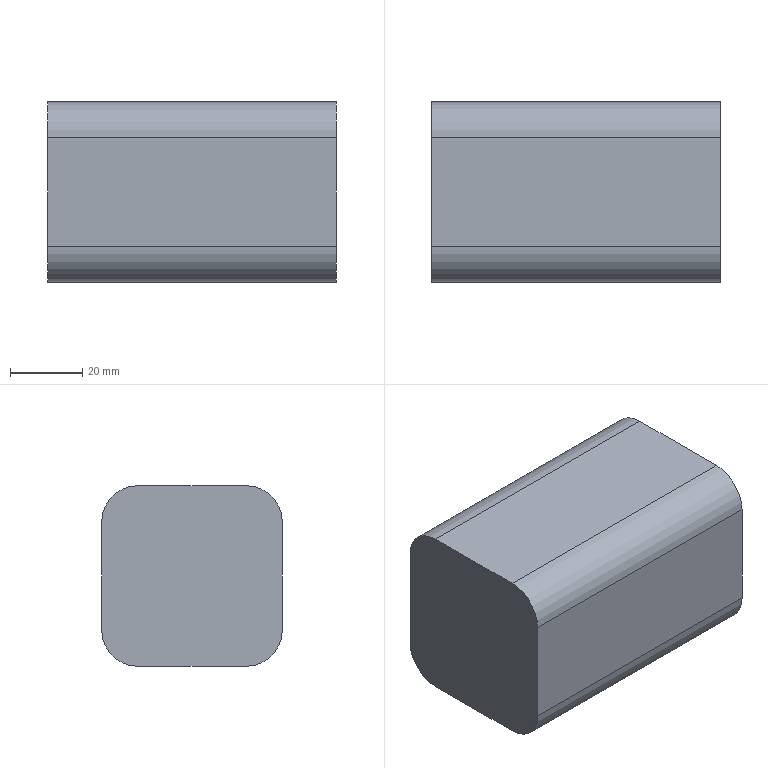Component | NX | MOTOR | 1 solid | 12 faces | box 80 x 50 x 50 mm | volume 187831 mm3 | plane 7 | cylinder 5 | commonest cylinder face diameters 20 x4 15 x1
STEP:
#1=CARTESIAN_POINT('',(0.,0.,0.));
#2=DIRECTION('',(0.,0.,1.));
#3=DIRECTION('',(1.,0.,0.));
#4=AXIS2_PLACEMENT_3D('',#1,#2,#3);
#5=CARTESIAN_POINT('',(213.574,526.538,-180.));
#6=VERTEX_POINT('',#5);
#7=CARTESIAN_POINT('',(213.574,526.538,-210.));
#8=VERTEX_POINT('',#7);
#9=CARTESIAN_POINT('',(213.574,526.538,-180.));
#10=DIRECTION('',(0.,0.,-1.));
#11=VECTOR('',#10,1.);
#12=LINE('',#9,#11);
#13=CARTESIAN_POINT('',(133.574,526.538,-180.));
#14=DIRECTION('',(0.,-1.,0.));
#15=DIRECTION('',(0.,0.,-1.));
#16=AXIS2_PLACEMENT_3D('',#13,#14,#15);
#17=PLANE('',#16);
#18=CARTESIAN_POINT('',(0.,80.));
#19=DIRECTION('',(1.,0.));
#20=VECTOR('',#19,1.);
#21=LINE('',#18,#20);
#22=(GEOMETRIC_REPRESENTATION_CONTEXT(2)PARAMETRIC_REPRESENTATION_CONTEXT()REPRESENTATION_CONTEXT('',''));
#23=DEFINITIONAL_REPRESENTATION('',(#21),#22);
#24=PCURVE('',#17,#23);
#25=CARTESIAN_POINT('',(213.574,516.538,-210.));
#26=DIRECTION('',(-1.,0.,0.));
#27=DIRECTION('',(0.,0.,-1.));
#28=AXIS2_PLACEMENT_3D('',#25,#26,#27);
#29=PLANE('',#28);
#30=CARTESIAN_POINT('',(-30.,-10.));
#31=DIRECTION('',(1.,0.));
#32=VECTOR('',#31,1.);
#33=LINE('',#30,#32);
#34=(GEOMETRIC_REPRESENTATION_CONTEXT(2)PARAMETRIC_REPRESENTATION_CONTEXT()REPRESENTATION_CONTEXT('',''));
#35=DEFINITIONAL_REPRESENTATION('',(#33),#34);
#36=PCURVE('',#29,#35);
#37=SURFACE_CURVE('',#12,(#24,#36),.PCURVE_S1.);
#38=EDGE_CURVE('',#6,#8,#37,.T.);
#39=ORIENTED_EDGE('',*,*,#38,.T.);
#40=CARTESIAN_POINT('',(133.574,526.538,-210.));
#41=VERTEX_POINT('',#40);
#42=CARTESIAN_POINT('',(133.574,526.538,-210.));
#43=DIRECTION('',(1.,0.,0.));
#44=VECTOR('',#43,1.);
#45=LINE('',#42,#44);
#46=CARTESIAN_POINT('',(30.,0.));
#47=DIRECTION('',(0.,1.));
#48=VECTOR('',#47,1.);
#49=LINE('',#46,#48);
#50=(GEOMETRIC_REPRESENTATION_CONTEXT(2)PARAMETRIC_REPRESENTATION_CONTEXT()REPRESENTATION_CONTEXT('',''));
#51=DEFINITIONAL_REPRESENTATION('',(#49),#50);
#52=PCURVE('',#17,#51);
#53=CARTESIAN_POINT('',(133.574,516.538,-210.));
#54=DIRECTION('',(1.,0.,0.));
#55=DIRECTION('',(0.,0.,1.));
#56=AXIS2_PLACEMENT_3D('',#53,#54,#55);
#57=CYLINDRICAL_SURFACE('',#56,10.);
#58=CARTESIAN_POINT('',(4.712,0.));
#59=DIRECTION('',(0.,1.));
#60=VECTOR('',#59,1.);
#61=LINE('',#58,#60);
#62=(GEOMETRIC_REPRESENTATION_CONTEXT(2)PARAMETRIC_REPRESENTATION_CONTEXT()REPRESENTATION_CONTEXT('',''));
#63=DEFINITIONAL_REPRESENTATION('',(#61),#62);
#64=PCURVE('',#57,#63);
#65=SURFACE_CURVE('',#45,(#52,#64),.PCURVE_S1.);
#66=EDGE_CURVE('',#41,#8,#65,.T.);
#67=ORIENTED_EDGE('',*,*,#66,.F.);
#68=CARTESIAN_POINT('',(133.574,526.538,-180.));
#69=VERTEX_POINT('',#68);
#70=CARTESIAN_POINT('',(133.574,526.538,-180.));
#71=DIRECTION('',(0.,0.,-1.));
#72=VECTOR('',#71,1.);
#73=LINE('',#70,#72);
#74=CARTESIAN_POINT('',(0.,0.));
#75=DIRECTION('',(1.,0.));
#76=VECTOR('',#75,1.);
#77=LINE('',#74,#76);
#78=(GEOMETRIC_REPRESENTATION_CONTEXT(2)PARAMETRIC_REPRESENTATION_CONTEXT()REPRESENTATION_CONTEXT('',''));
#79=DEFINITIONAL_REPRESENTATION('',(#77),#78);
#80=PCURVE('',#17,#79);
#81=CARTESIAN_POINT('',(133.574,516.538,-210.));
#82=DIRECTION('',(-1.,0.,0.));
#83=DIRECTION('',(0.,0.,-1.));
#84=AXIS2_PLACEMENT_3D('',#81,#82,#83);
#85=PLANE('',#84);
#86=CARTESIAN_POINT('',(-30.,-10.));
#87=DIRECTION('',(1.,0.));
#88=VECTOR('',#87,1.);
#89=LINE('',#86,#88);
#90=(GEOMETRIC_REPRESENTATION_CONTEXT(2)PARAMETRIC_REPRESENTATION_CONTEXT()REPRESENTATION_CONTEXT('',''));
#91=DEFINITIONAL_REPRESENTATION('',(#89),#90);
#92=PCURVE('',#85,#91);
#93=SURFACE_CURVE('',#73,(#80,#92),.PCURVE_S1.);
#94=EDGE_CURVE('',#69,#41,#93,.T.);
#95=ORIENTED_EDGE('',*,*,#94,.F.);
#96=CARTESIAN_POINT('',(133.574,526.538,-180.));
#97=DIRECTION('',(1.,0.,0.));
#98=VECTOR('',#97,1.);
#99=LINE('',#96,#98);
#100=CARTESIAN_POINT('',(0.,0.));
#101=DIRECTION('',(0.,1.));
#102=VECTOR('',#101,1.);
#103=LINE('',#100,#102);
#104=(GEOMETRIC_REPRESENTATION_CONTEXT(2)PARAMETRIC_REPRESENTATION_CONTEXT()REPRESENTATION_CONTEXT('',''));
#105=DEFINITIONAL_REPRESENTATION('',(#103),#104);
#106=PCURVE('',#17,#105);
#107=CARTESIAN_POINT('',(133.574,516.538,-180.));
#108=DIRECTION('',(1.,0.,0.));
#109=DIRECTION('',(0.,0.,1.));
#110=AXIS2_PLACEMENT_3D('',#107,#108,#109);
#111=CYLINDRICAL_SURFACE('',#110,10.);
#112=CARTESIAN_POINT('',(4.712,0.));
#113=DIRECTION('',(0.,1.));
#114=VECTOR('',#113,1.);
#115=LINE('',#112,#114);
#116=(GEOMETRIC_REPRESENTATION_CONTEXT(2)PARAMETRIC_REPRESENTATION_CONTEXT()REPRESENTATION_CONTEXT('',''));
#117=DEFINITIONAL_REPRESENTATION('',(#115),#116);
#118=PCURVE('',#111,#117);
#119=SURFACE_CURVE('',#99,(#106,#118),.PCURVE_S1.);
#120=EDGE_CURVE('',#69,#6,#119,.T.);
#121=ORIENTED_EDGE('',*,*,#120,.T.);
#122=EDGE_LOOP('',(#39,#67,#95,#121));
#123=FACE_BOUND('',#122,.T.);
#124=ADVANCED_FACE('',(#123),#17,.F.);
#125=CARTESIAN_POINT('',(213.574,516.538,-220.));
#126=VERTEX_POINT('',#125);
#127=CARTESIAN_POINT('',(213.574,516.538,-210.));
#128=DIRECTION('',(-1.,0.,0.));
#129=DIRECTION('',(0.,-1.,0.));
#130=AXIS2_PLACEMENT_3D('',#127,#128,#129);
#131=CIRCLE('',#130,10.);
#132=CARTESIAN_POINT('',(7.854,80.));
#133=DIRECTION('',(-1.,0.));
#134=VECTOR('',#133,1.);
#135=LINE('',#132,#134);
#136=(GEOMETRIC_REPRESENTATION_CONTEXT(2)PARAMETRIC_REPRESENTATION_CONTEXT()REPRESENTATION_CONTEXT('',''));
#137=DEFINITIONAL_REPRESENTATION('',(#135),#136);
#138=PCURVE('',#57,#137);
#139=CARTESIAN_POINT('',(0.,0.));
#140=DIRECTION('',(0.,1.));
#141=AXIS2_PLACEMENT_2D('',#139,#140);
#142=CIRCLE('',#141,10.);
#143=(GEOMETRIC_REPRESENTATION_CONTEXT(2)PARAMETRIC_REPRESENTATION_CONTEXT()REPRESENTATION_CONTEXT('',''));
#144=DEFINITIONAL_REPRESENTATION('',(#142),#143);
#145=PCURVE('',#29,#144);
#146=SURFACE_CURVE('',#131,(#138,#145),.PCURVE_S1.);
#147=EDGE_CURVE('',#8,#126,#146,.T.);
#148=ORIENTED_EDGE('',*,*,#147,.T.);
#149=CARTESIAN_POINT('',(133.574,516.538,-220.));
#150=VERTEX_POINT('',#149);
#151=CARTESIAN_POINT('',(133.574,516.538,-220.));
#152=DIRECTION('',(1.,0.,0.));
#153=VECTOR('',#152,1.);
#154=LINE('',#151,#153);
#155=CARTESIAN_POINT('',(3.142,0.));
#156=DIRECTION('',(0.,1.));
#157=VECTOR('',#156,1.);
#158=LINE('',#155,#157);
#159=(GEOMETRIC_REPRESENTATION_CONTEXT(2)PARAMETRIC_REPRESENTATION_CONTEXT()REPRESENTATION_CONTEXT('',''));
#160=DEFINITIONAL_REPRESENTATION('',(#158),#159);
#161=PCURVE('',#57,#160);
#162=CARTESIAN_POINT('',(133.574,516.538,-220.));
#163=DIRECTION('',(0.,-0.,1.));
#164=DIRECTION('',(0.,-1.,-0.));
#165=AXIS2_PLACEMENT_3D('',#162,#163,#164);
#166=PLANE('',#165);
#167=CARTESIAN_POINT('',(0.,0.));
#168=DIRECTION('',(0.,1.));
#169=VECTOR('',#168,1.);
#170=LINE('',#167,#169);
#171=(GEOMETRIC_REPRESENTATION_CONTEXT(2)PARAMETRIC_REPRESENTATION_CONTEXT()REPRESENTATION_CONTEXT('',''));
#172=DEFINITIONAL_REPRESENTATION('',(#170),#171);
#173=PCURVE('',#166,#172);
#174=SURFACE_CURVE('',#154,(#161,#173),.PCURVE_S1.);
#175=EDGE_CURVE('',#150,#126,#174,.T.);
#176=ORIENTED_EDGE('',*,*,#175,.F.);
#177=CARTESIAN_POINT('',(133.574,516.538,-210.));
#178=DIRECTION('',(-1.,0.,0.));
#179=DIRECTION('',(0.,-1.,0.));
#180=AXIS2_PLACEMENT_3D('',#177,#178,#179);
#181=CIRCLE('',#180,10.);
#182=CARTESIAN_POINT('',(7.854,0.));
#183=DIRECTION('',(-1.,0.));
#184=VECTOR('',#183,1.);
#185=LINE('',#182,#184);
#186=(GEOMETRIC_REPRESENTATION_CONTEXT(2)PARAMETRIC_REPRESENTATION_CONTEXT()REPRESENTATION_CONTEXT('',''));
#187=DEFINITIONAL_REPRESENTATION('',(#185),#186);
#188=PCURVE('',#57,#187);
#189=CARTESIAN_POINT('',(0.,0.));
#190=DIRECTION('',(0.,1.));
#191=AXIS2_PLACEMENT_2D('',#189,#190);
#192=CIRCLE('',#191,10.);
#193=(GEOMETRIC_REPRESENTATION_CONTEXT(2)PARAMETRIC_REPRESENTATION_CONTEXT()REPRESENTATION_CONTEXT('',''));
#194=DEFINITIONAL_REPRESENTATION('',(#192),#193);
#195=PCURVE('',#85,#194);
#196=SURFACE_CURVE('',#181,(#188,#195),.PCURVE_S1.);
#197=EDGE_CURVE('',#41,#150,#196,.T.);
#198=ORIENTED_EDGE('',*,*,#197,.F.);
#199=ORIENTED_EDGE('',*,*,#66,.T.);
#200=EDGE_LOOP('',(#148,#176,#198,#199));
#201=FACE_BOUND('',#200,.T.);
#202=ADVANCED_FACE('',(#201),#57,.T.);
#203=CARTESIAN_POINT('',(213.574,486.538,-220.));
#204=VERTEX_POINT('',#203);
#205=CARTESIAN_POINT('',(213.574,516.538,-220.));
#206=DIRECTION('',(0.,-1.,-0.));
#207=VECTOR('',#206,1.);
#208=LINE('',#205,#207);
#209=CARTESIAN_POINT('',(0.,80.));
#210=DIRECTION('',(1.,0.));
#211=VECTOR('',#210,1.);
#212=LINE('',#209,#211);
#213=(GEOMETRIC_REPRESENTATION_CONTEXT(2)PARAMETRIC_REPRESENTATION_CONTEXT()REPRESENTATION_CONTEXT('',''));
#214=DEFINITIONAL_REPRESENTATION('',(#212),#213);
#215=PCURVE('',#166,#214);
#216=CARTESIAN_POINT('',(10.,0.));
#217=DIRECTION('',(0.,1.));
#218=VECTOR('',#217,1.);
#219=LINE('',#216,#218);
#220=(GEOMETRIC_REPRESENTATION_CONTEXT(2)PARAMETRIC_REPRESENTATION_CONTEXT()REPRESENTATION_CONTEXT('',''));
#221=DEFINITIONAL_REPRESENTATION('',(#219),#220);
#222=PCURVE('',#29,#221);
#223=SURFACE_CURVE('',#208,(#215,#222),.PCURVE_S1.);
#224=EDGE_CURVE('',#126,#204,#223,.T.);
#225=ORIENTED_EDGE('',*,*,#224,.T.);
#226=CARTESIAN_POINT('',(133.574,486.538,-220.));
#227=VERTEX_POINT('',#226);
#228=CARTESIAN_POINT('',(133.574,486.538,-220.));
#229=DIRECTION('',(1.,0.,0.));
#230=VECTOR('',#229,1.);
#231=LINE('',#228,#230);
#232=CARTESIAN_POINT('',(30.,0.));
#233=DIRECTION('',(0.,1.));
#234=VECTOR('',#233,1.);
#235=LINE('',#232,#234);
#236=(GEOMETRIC_REPRESENTATION_CONTEXT(2)PARAMETRIC_REPRESENTATION_CONTEXT()REPRESENTATION_CONTEXT('',''));
#237=DEFINITIONAL_REPRESENTATION('',(#235),#236);
#238=PCURVE('',#166,#237);
#239=CARTESIAN_POINT('',(133.574,486.538,-210.));
#240=DIRECTION('',(1.,0.,0.));
#241=DIRECTION('',(0.,0.,1.));
#242=AXIS2_PLACEMENT_3D('',#239,#240,#241);
#243=CYLINDRICAL_SURFACE('',#242,10.);
#244=CARTESIAN_POINT('',(3.142,0.));
#245=DIRECTION('',(0.,1.));
#246=VECTOR('',#245,1.);
#247=LINE('',#244,#246);
#248=(GEOMETRIC_REPRESENTATION_CONTEXT(2)PARAMETRIC_REPRESENTATION_CONTEXT()REPRESENTATION_CONTEXT('',''));
#249=DEFINITIONAL_REPRESENTATION('',(#247),#248);
#250=PCURVE('',#243,#249);
#251=SURFACE_CURVE('',#231,(#238,#250),.PCURVE_S1.);
#252=EDGE_CURVE('',#227,#204,#251,.T.);
#253=ORIENTED_EDGE('',*,*,#252,.F.);
#254=CARTESIAN_POINT('',(133.574,516.538,-220.));
#255=DIRECTION('',(0.,-1.,-0.));
#256=VECTOR('',#255,1.);
#257=LINE('',#254,#256);
#258=CARTESIAN_POINT('',(0.,0.));
#259=DIRECTION('',(1.,0.));
#260=VECTOR('',#259,1.);
#261=LINE('',#258,#260);
#262=(GEOMETRIC_REPRESENTATION_CONTEXT(2)PARAMETRIC_REPRESENTATION_CONTEXT()REPRESENTATION_CONTEXT('',''));
#263=DEFINITIONAL_REPRESENTATION('',(#261),#262);
#264=PCURVE('',#166,#263);
#265=CARTESIAN_POINT('',(10.,0.));
#266=DIRECTION('',(0.,1.));
#267=VECTOR('',#266,1.);
#268=LINE('',#265,#267);
#269=(GEOMETRIC_REPRESENTATION_CONTEXT(2)PARAMETRIC_REPRESENTATION_CONTEXT()REPRESENTATION_CONTEXT('',''));
#270=DEFINITIONAL_REPRESENTATION('',(#268),#269);
#271=PCURVE('',#85,#270);
#272=SURFACE_CURVE('',#257,(#264,#271),.PCURVE_S1.);
#273=EDGE_CURVE('',#150,#227,#272,.T.);
#274=ORIENTED_EDGE('',*,*,#273,.F.);
#275=ORIENTED_EDGE('',*,*,#175,.T.);
#276=EDGE_LOOP('',(#225,#253,#274,#275));
#277=FACE_BOUND('',#276,.T.);
#278=ADVANCED_FACE('',(#277),#166,.F.);
#279=CARTESIAN_POINT('',(213.574,476.538,-210.));
#280=VERTEX_POINT('',#279);
#281=CARTESIAN_POINT('',(213.574,486.538,-210.));
#282=DIRECTION('',(-1.,0.,0.));
#283=DIRECTION('',(0.,-1.,0.));
#284=AXIS2_PLACEMENT_3D('',#281,#282,#283);
#285=CIRCLE('',#284,10.);
#286=CARTESIAN_POINT('',(7.854,80.));
#287=DIRECTION('',(-1.,0.));
#288=VECTOR('',#287,1.);
#289=LINE('',#286,#288);
#290=(GEOMETRIC_REPRESENTATION_CONTEXT(2)PARAMETRIC_REPRESENTATION_CONTEXT()REPRESENTATION_CONTEXT('',''));
#291=DEFINITIONAL_REPRESENTATION('',(#289),#290);
#292=PCURVE('',#243,#291);
#293=CARTESIAN_POINT('',(0.,30.));
#294=DIRECTION('',(0.,1.));
#295=AXIS2_PLACEMENT_2D('',#293,#294);
#296=CIRCLE('',#295,10.);
#297=(GEOMETRIC_REPRESENTATION_CONTEXT(2)PARAMETRIC_REPRESENTATION_CONTEXT()REPRESENTATION_CONTEXT('',''));
#298=DEFINITIONAL_REPRESENTATION('',(#296),#297);
#299=PCURVE('',#29,#298);
#300=SURFACE_CURVE('',#285,(#292,#299),.PCURVE_S1.);
#301=EDGE_CURVE('',#204,#280,#300,.T.);
#302=ORIENTED_EDGE('',*,*,#301,.T.);
#303=CARTESIAN_POINT('',(133.574,476.538,-210.));
#304=VERTEX_POINT('',#303);
#305=CARTESIAN_POINT('',(133.574,476.538,-210.));
#306=DIRECTION('',(1.,0.,0.));
#307=VECTOR('',#306,1.);
#308=LINE('',#305,#307);
#309=CARTESIAN_POINT('',(1.571,0.));
#310=DIRECTION('',(0.,1.));
#311=VECTOR('',#310,1.);
#312=LINE('',#309,#311);
#313=(GEOMETRIC_REPRESENTATION_CONTEXT(2)PARAMETRIC_REPRESENTATION_CONTEXT()REPRESENTATION_CONTEXT('',''));
#314=DEFINITIONAL_REPRESENTATION('',(#312),#313);
#315=PCURVE('',#243,#314);
#316=CARTESIAN_POINT('',(133.574,476.538,-210.));
#317=DIRECTION('',(0.,1.,0.));
#318=DIRECTION('',(0.,0.,1.));
#319=AXIS2_PLACEMENT_3D('',#316,#317,#318);
#320=PLANE('',#319);
#321=CARTESIAN_POINT('',(0.,0.));
#322=DIRECTION('',(0.,1.));
#323=VECTOR('',#322,1.);
#324=LINE('',#321,#323);
#325=(GEOMETRIC_REPRESENTATION_CONTEXT(2)PARAMETRIC_REPRESENTATION_CONTEXT()REPRESENTATION_CONTEXT('',''));
#326=DEFINITIONAL_REPRESENTATION('',(#324),#325);
#327=PCURVE('',#320,#326);
#328=SURFACE_CURVE('',#308,(#315,#327),.PCURVE_S1.);
#329=EDGE_CURVE('',#304,#280,#328,.T.);
#330=ORIENTED_EDGE('',*,*,#329,.F.);
#331=CARTESIAN_POINT('',(133.574,486.538,-210.));
#332=DIRECTION('',(-1.,0.,0.));
#333=DIRECTION('',(0.,-1.,0.));
#334=AXIS2_PLACEMENT_3D('',#331,#332,#333);
#335=CIRCLE('',#334,10.);
#336=CARTESIAN_POINT('',(7.854,0.));
#337=DIRECTION('',(-1.,0.));
#338=VECTOR('',#337,1.);
#339=LINE('',#336,#338);
#340=(GEOMETRIC_REPRESENTATION_CONTEXT(2)PARAMETRIC_REPRESENTATION_CONTEXT()REPRESENTATION_CONTEXT('',''));
#341=DEFINITIONAL_REPRESENTATION('',(#339),#340);
#342=PCURVE('',#243,#341);
#343=CARTESIAN_POINT('',(0.,30.));
#344=DIRECTION('',(0.,1.));
#345=AXIS2_PLACEMENT_2D('',#343,#344);
#346=CIRCLE('',#345,10.);
#347=(GEOMETRIC_REPRESENTATION_CONTEXT(2)PARAMETRIC_REPRESENTATION_CONTEXT()REPRESENTATION_CONTEXT('',''));
#348=DEFINITIONAL_REPRESENTATION('',(#346),#347);
#349=PCURVE('',#85,#348);
#350=SURFACE_CURVE('',#335,(#342,#349),.PCURVE_S1.);
#351=EDGE_CURVE('',#227,#304,#350,.T.);
#352=ORIENTED_EDGE('',*,*,#351,.F.);
#353=ORIENTED_EDGE('',*,*,#252,.T.);
#354=EDGE_LOOP('',(#302,#330,#352,#353));
#355=FACE_BOUND('',#354,.T.);
#356=ADVANCED_FACE('',(#355),#243,.T.);
#357=CARTESIAN_POINT('',(213.574,476.538,-180.));
#358=VERTEX_POINT('',#357);
#359=CARTESIAN_POINT('',(213.574,476.538,-210.));
#360=DIRECTION('',(0.,0.,1.));
#361=VECTOR('',#360,1.);
#362=LINE('',#359,#361);
#363=CARTESIAN_POINT('',(0.,80.));
#364=DIRECTION('',(1.,0.));
#365=VECTOR('',#364,1.);
#366=LINE('',#363,#365);
#367=(GEOMETRIC_REPRESENTATION_CONTEXT(2)PARAMETRIC_REPRESENTATION_CONTEXT()REPRESENTATION_CONTEXT('',''));
#368=DEFINITIONAL_REPRESENTATION('',(#366),#367);
#369=PCURVE('',#320,#368);
#370=CARTESIAN_POINT('',(0.,40.));
#371=DIRECTION('',(-1.,0.));
#372=VECTOR('',#371,1.);
#373=LINE('',#370,#372);
#374=(GEOMETRIC_REPRESENTATION_CONTEXT(2)PARAMETRIC_REPRESENTATION_CONTEXT()REPRESENTATION_CONTEXT('',''));
#375=DEFINITIONAL_REPRESENTATION('',(#373),#374);
#376=PCURVE('',#29,#375);
#377=SURFACE_CURVE('',#362,(#369,#376),.PCURVE_S1.);
#378=EDGE_CURVE('',#280,#358,#377,.T.);
#379=ORIENTED_EDGE('',*,*,#378,.T.);
#380=CARTESIAN_POINT('',(133.574,476.538,-180.));
#381=VERTEX_POINT('',#380);
#382=CARTESIAN_POINT('',(133.574,476.538,-180.));
#383=DIRECTION('',(1.,0.,0.));
#384=VECTOR('',#383,1.);
#385=LINE('',#382,#384);
#386=CARTESIAN_POINT('',(30.,0.));
#387=DIRECTION('',(0.,1.));
#388=VECTOR('',#387,1.);
#389=LINE('',#386,#388);
#390=(GEOMETRIC_REPRESENTATION_CONTEXT(2)PARAMETRIC_REPRESENTATION_CONTEXT()REPRESENTATION_CONTEXT('',''));
#391=DEFINITIONAL_REPRESENTATION('',(#389),#390);
#392=PCURVE('',#320,#391);
#393=CARTESIAN_POINT('',(133.574,486.538,-180.));
#394=DIRECTION('',(1.,0.,0.));
#395=DIRECTION('',(0.,0.,1.));
#396=AXIS2_PLACEMENT_3D('',#393,#394,#395);
#397=CYLINDRICAL_SURFACE('',#396,10.);
#398=CARTESIAN_POINT('',(1.571,0.));
#399=DIRECTION('',(0.,1.));
#400=VECTOR('',#399,1.);
#401=LINE('',#398,#400);
#402=(GEOMETRIC_REPRESENTATION_CONTEXT(2)PARAMETRIC_REPRESENTATION_CONTEXT()REPRESENTATION_CONTEXT('',''));
#403=DEFINITIONAL_REPRESENTATION('',(#401),#402);
#404=PCURVE('',#397,#403);
#405=SURFACE_CURVE('',#385,(#392,#404),.PCURVE_S1.);
#406=EDGE_CURVE('',#381,#358,#405,.T.);
#407=ORIENTED_EDGE('',*,*,#406,.F.);
#408=CARTESIAN_POINT('',(133.574,476.538,-210.));
#409=DIRECTION('',(0.,0.,1.));
#410=VECTOR('',#409,1.);
#411=LINE('',#408,#410);
#412=CARTESIAN_POINT('',(0.,0.));
#413=DIRECTION('',(1.,0.));
#414=VECTOR('',#413,1.);
#415=LINE('',#412,#414);
#416=(GEOMETRIC_REPRESENTATION_CONTEXT(2)PARAMETRIC_REPRESENTATION_CONTEXT()REPRESENTATION_CONTEXT('',''));
#417=DEFINITIONAL_REPRESENTATION('',(#415),#416);
#418=PCURVE('',#320,#417);
#419=CARTESIAN_POINT('',(0.,40.));
#420=DIRECTION('',(-1.,0.));
#421=VECTOR('',#420,1.);
#422=LINE('',#419,#421);
#423=(GEOMETRIC_REPRESENTATION_CONTEXT(2)PARAMETRIC_REPRESENTATION_CONTEXT()REPRESENTATION_CONTEXT('',''));
#424=DEFINITIONAL_REPRESENTATION('',(#422),#423);
#425=PCURVE('',#85,#424);
#426=SURFACE_CURVE('',#411,(#418,#425),.PCURVE_S1.);
#427=EDGE_CURVE('',#304,#381,#426,.T.);
#428=ORIENTED_EDGE('',*,*,#427,.F.);
#429=ORIENTED_EDGE('',*,*,#329,.T.);
#430=EDGE_LOOP('',(#379,#407,#428,#429));
#431=FACE_BOUND('',#430,.T.);
#432=ADVANCED_FACE('',(#431),#320,.F.);
#433=CARTESIAN_POINT('',(213.574,486.538,-170.));
#434=VERTEX_POINT('',#433);
#435=CARTESIAN_POINT('',(213.574,486.538,-180.));
#436=DIRECTION('',(-1.,0.,0.));
#437=DIRECTION('',(0.,-1.,0.));
#438=AXIS2_PLACEMENT_3D('',#435,#436,#437);
#439=CIRCLE('',#438,10.);
#440=CARTESIAN_POINT('',(1.571,80.));
#441=DIRECTION('',(-1.,0.));
#442=VECTOR('',#441,1.);
#443=LINE('',#440,#442);
#444=(GEOMETRIC_REPRESENTATION_CONTEXT(2)PARAMETRIC_REPRESENTATION_CONTEXT()REPRESENTATION_CONTEXT('',''));
#445=DEFINITIONAL_REPRESENTATION('',(#443),#444);
#446=PCURVE('',#397,#445);
#447=CARTESIAN_POINT('',(-30.,30.));
#448=DIRECTION('',(0.,1.));
#449=AXIS2_PLACEMENT_2D('',#447,#448);
#450=CIRCLE('',#449,10.);
#451=(GEOMETRIC_REPRESENTATION_CONTEXT(2)PARAMETRIC_REPRESENTATION_CONTEXT()REPRESENTATION_CONTEXT('',''));
#452=DEFINITIONAL_REPRESENTATION('',(#450),#451);
#453=PCURVE('',#29,#452);
#454=SURFACE_CURVE('',#439,(#446,#453),.PCURVE_S1.);
#455=EDGE_CURVE('',#358,#434,#454,.T.);
#456=ORIENTED_EDGE('',*,*,#455,.T.);
#457=CARTESIAN_POINT('',(133.574,486.538,-170.));
#458=VERTEX_POINT('',#457);
#459=CARTESIAN_POINT('',(133.574,486.538,-170.));
#460=DIRECTION('',(1.,0.,0.));
#461=VECTOR('',#460,1.);
#462=LINE('',#459,#461);
#463=CARTESIAN_POINT('',(0.,0.));
#464=DIRECTION('',(0.,1.));
#465=VECTOR('',#464,1.);
#466=LINE('',#463,#465);
#467=(GEOMETRIC_REPRESENTATION_CONTEXT(2)PARAMETRIC_REPRESENTATION_CONTEXT()REPRESENTATION_CONTEXT('',''));
#468=DEFINITIONAL_REPRESENTATION('',(#466),#467);
#469=PCURVE('',#397,#468);
#470=CARTESIAN_POINT('',(133.574,486.538,-170.));
#471=DIRECTION('',(0.,-0.,-1.));
#472=DIRECTION('',(0.,1.,-0.));
#473=AXIS2_PLACEMENT_3D('',#470,#471,#472);
#474=PLANE('',#473);
#475=CARTESIAN_POINT('',(0.,0.));
#476=DIRECTION('',(0.,1.));
#477=VECTOR('',#476,1.);
#478=LINE('',#475,#477);
#479=(GEOMETRIC_REPRESENTATION_CONTEXT(2)PARAMETRIC_REPRESENTATION_CONTEXT()REPRESENTATION_CONTEXT('',''));
#480=DEFINITIONAL_REPRESENTATION('',(#478),#479);
#481=PCURVE('',#474,#480);
#482=SURFACE_CURVE('',#462,(#469,#481),.PCURVE_S1.);
#483=EDGE_CURVE('',#458,#434,#482,.T.);
#484=ORIENTED_EDGE('',*,*,#483,.F.);
#485=CARTESIAN_POINT('',(133.574,486.538,-180.));
#486=DIRECTION('',(-1.,0.,0.));
#487=DIRECTION('',(0.,-1.,0.));
#488=AXIS2_PLACEMENT_3D('',#485,#486,#487);
#489=CIRCLE('',#488,10.);
#490=CARTESIAN_POINT('',(1.571,0.));
#491=DIRECTION('',(-1.,0.));
#492=VECTOR('',#491,1.);
#493=LINE('',#490,#492);
#494=(GEOMETRIC_REPRESENTATION_CONTEXT(2)PARAMETRIC_REPRESENTATION_CONTEXT()REPRESENTATION_CONTEXT('',''));
#495=DEFINITIONAL_REPRESENTATION('',(#493),#494);
#496=PCURVE('',#397,#495);
#497=CARTESIAN_POINT('',(-30.,30.));
#498=DIRECTION('',(0.,1.));
#499=AXIS2_PLACEMENT_2D('',#497,#498);
#500=CIRCLE('',#499,10.);
#501=(GEOMETRIC_REPRESENTATION_CONTEXT(2)PARAMETRIC_REPRESENTATION_CONTEXT()REPRESENTATION_CONTEXT('',''));
#502=DEFINITIONAL_REPRESENTATION('',(#500),#501);
#503=PCURVE('',#85,#502);
#504=SURFACE_CURVE('',#489,(#496,#503),.PCURVE_S1.);
#505=EDGE_CURVE('',#381,#458,#504,.T.);
#506=ORIENTED_EDGE('',*,*,#505,.F.);
#507=ORIENTED_EDGE('',*,*,#406,.T.);
#508=EDGE_LOOP('',(#456,#484,#506,#507));
#509=FACE_BOUND('',#508,.T.);
#510=ADVANCED_FACE('',(#509),#397,.T.);
#511=CARTESIAN_POINT('',(213.574,516.538,-170.));
#512=VERTEX_POINT('',#511);
#513=CARTESIAN_POINT('',(213.574,486.538,-170.));
#514=DIRECTION('',(0.,1.,-0.));
#515=VECTOR('',#514,1.);
#516=LINE('',#513,#515);
#517=CARTESIAN_POINT('',(0.,80.));
#518=DIRECTION('',(1.,0.));
#519=VECTOR('',#518,1.);
#520=LINE('',#517,#519);
#521=(GEOMETRIC_REPRESENTATION_CONTEXT(2)PARAMETRIC_REPRESENTATION_CONTEXT()REPRESENTATION_CONTEXT('',''));
#522=DEFINITIONAL_REPRESENTATION('',(#520),#521);
#523=PCURVE('',#474,#522);
#524=CARTESIAN_POINT('',(-40.,30.));
#525=DIRECTION('',(0.,-1.));
#526=VECTOR('',#525,1.);
#527=LINE('',#524,#526);
#528=(GEOMETRIC_REPRESENTATION_CONTEXT(2)PARAMETRIC_REPRESENTATION_CONTEXT()REPRESENTATION_CONTEXT('',''));
#529=DEFINITIONAL_REPRESENTATION('',(#527),#528);
#530=PCURVE('',#29,#529);
#531=SURFACE_CURVE('',#516,(#523,#530),.PCURVE_S1.);
#532=EDGE_CURVE('',#434,#512,#531,.T.);
#533=ORIENTED_EDGE('',*,*,#532,.T.);
#534=CARTESIAN_POINT('',(133.574,516.538,-170.));
#535=VERTEX_POINT('',#534);
#536=CARTESIAN_POINT('',(133.574,516.538,-170.));
#537=DIRECTION('',(1.,0.,0.));
#538=VECTOR('',#537,1.);
#539=LINE('',#536,#538);
#540=CARTESIAN_POINT('',(30.,0.));
#541=DIRECTION('',(0.,1.));
#542=VECTOR('',#541,1.);
#543=LINE('',#540,#542);
#544=(GEOMETRIC_REPRESENTATION_CONTEXT(2)PARAMETRIC_REPRESENTATION_CONTEXT()REPRESENTATION_CONTEXT('',''));
#545=DEFINITIONAL_REPRESENTATION('',(#543),#544);
#546=PCURVE('',#474,#545);
#547=CARTESIAN_POINT('',(6.283,0.));
#548=DIRECTION('',(0.,1.));
#549=VECTOR('',#548,1.);
#550=LINE('',#547,#549);
#551=(GEOMETRIC_REPRESENTATION_CONTEXT(2)PARAMETRIC_REPRESENTATION_CONTEXT()REPRESENTATION_CONTEXT('',''));
#552=DEFINITIONAL_REPRESENTATION('',(#550),#551);
#553=PCURVE('',#111,#552);
#554=SURFACE_CURVE('',#539,(#546,#553),.PCURVE_S1.);
#555=EDGE_CURVE('',#535,#512,#554,.T.);
#556=ORIENTED_EDGE('',*,*,#555,.F.);
#557=CARTESIAN_POINT('',(133.574,486.538,-170.));
#558=DIRECTION('',(0.,1.,-0.));
#559=VECTOR('',#558,1.);
#560=LINE('',#557,#559);
#561=CARTESIAN_POINT('',(0.,0.));
#562=DIRECTION('',(1.,0.));
#563=VECTOR('',#562,1.);
#564=LINE('',#561,#563);
#565=(GEOMETRIC_REPRESENTATION_CONTEXT(2)PARAMETRIC_REPRESENTATION_CONTEXT()REPRESENTATION_CONTEXT('',''));
#566=DEFINITIONAL_REPRESENTATION('',(#564),#565);
#567=PCURVE('',#474,#566);
#568=CARTESIAN_POINT('',(-40.,30.));
#569=DIRECTION('',(0.,-1.));
#570=VECTOR('',#569,1.);
#571=LINE('',#568,#570);
#572=(GEOMETRIC_REPRESENTATION_CONTEXT(2)PARAMETRIC_REPRESENTATION_CONTEXT()REPRESENTATION_CONTEXT('',''));
#573=DEFINITIONAL_REPRESENTATION('',(#571),#572);
#574=PCURVE('',#85,#573);
#575=SURFACE_CURVE('',#560,(#567,#574),.PCURVE_S1.);
#576=EDGE_CURVE('',#458,#535,#575,.T.);
#577=ORIENTED_EDGE('',*,*,#576,.F.);
#578=ORIENTED_EDGE('',*,*,#483,.T.);
#579=EDGE_LOOP('',(#533,#556,#577,#578));
#580=FACE_BOUND('',#579,.T.);
#581=ADVANCED_FACE('',(#580),#474,.F.);
#582=CARTESIAN_POINT('',(213.574,516.538,-180.));
#583=DIRECTION('',(-1.,0.,0.));
#584=DIRECTION('',(0.,-1.,0.));
#585=AXIS2_PLACEMENT_3D('',#582,#583,#584);
#586=CIRCLE('',#585,10.);
#587=CARTESIAN_POINT('',(7.854,80.));
#588=DIRECTION('',(-1.,0.));
#589=VECTOR('',#588,1.);
#590=LINE('',#587,#589);
#591=(GEOMETRIC_REPRESENTATION_CONTEXT(2)PARAMETRIC_REPRESENTATION_CONTEXT()REPRESENTATION_CONTEXT('',''));
#592=DEFINITIONAL_REPRESENTATION('',(#590),#591);
#593=PCURVE('',#111,#592);
#594=CARTESIAN_POINT('',(-30.,0.));
#595=DIRECTION('',(0.,1.));
#596=AXIS2_PLACEMENT_2D('',#594,#595);
#597=CIRCLE('',#596,10.);
#598=(GEOMETRIC_REPRESENTATION_CONTEXT(2)PARAMETRIC_REPRESENTATION_CONTEXT()REPRESENTATION_CONTEXT('',''));
#599=DEFINITIONAL_REPRESENTATION('',(#597),#598);
#600=PCURVE('',#29,#599);
#601=SURFACE_CURVE('',#586,(#593,#600),.PCURVE_S1.);
#602=EDGE_CURVE('',#512,#6,#601,.T.);
#603=ORIENTED_EDGE('',*,*,#602,.T.);
#604=ORIENTED_EDGE('',*,*,#120,.F.);
#605=CARTESIAN_POINT('',(133.574,516.538,-180.));
#606=DIRECTION('',(-1.,0.,0.));
#607=DIRECTION('',(0.,-1.,0.));
#608=AXIS2_PLACEMENT_3D('',#605,#606,#607);
#609=CIRCLE('',#608,10.);
#610=CARTESIAN_POINT('',(7.854,0.));
#611=DIRECTION('',(-1.,0.));
#612=VECTOR('',#611,1.);
#613=LINE('',#610,#612);
#614=(GEOMETRIC_REPRESENTATION_CONTEXT(2)PARAMETRIC_REPRESENTATION_CONTEXT()REPRESENTATION_CONTEXT('',''));
#615=DEFINITIONAL_REPRESENTATION('',(#613),#614);
#616=PCURVE('',#111,#615);
#617=CARTESIAN_POINT('',(-30.,0.));
#618=DIRECTION('',(0.,1.));
#619=AXIS2_PLACEMENT_2D('',#617,#618);
#620=CIRCLE('',#619,10.);
#621=(GEOMETRIC_REPRESENTATION_CONTEXT(2)PARAMETRIC_REPRESENTATION_CONTEXT()REPRESENTATION_CONTEXT('',''));
#622=DEFINITIONAL_REPRESENTATION('',(#620),#621);
#623=PCURVE('',#85,#622);
#624=SURFACE_CURVE('',#609,(#616,#623),.PCURVE_S1.);
#625=EDGE_CURVE('',#535,#69,#624,.T.);
#626=ORIENTED_EDGE('',*,*,#625,.F.);
#627=ORIENTED_EDGE('',*,*,#555,.T.);
#628=EDGE_LOOP('',(#603,#604,#626,#627));
#629=FACE_BOUND('',#628,.T.);
#630=ADVANCED_FACE('',(#629),#111,.T.);
#631=ORIENTED_EDGE('',*,*,#94,.T.);
#632=ORIENTED_EDGE('',*,*,#197,.T.);
#633=ORIENTED_EDGE('',*,*,#273,.T.);
#634=ORIENTED_EDGE('',*,*,#351,.T.);
#635=ORIENTED_EDGE('',*,*,#427,.T.);
#636=ORIENTED_EDGE('',*,*,#505,.T.);
#637=ORIENTED_EDGE('',*,*,#576,.T.);
#638=ORIENTED_EDGE('',*,*,#625,.T.);
#639=EDGE_LOOP('',(#631,#632,#633,#634,#635,#636,#637,#638));
#640=FACE_BOUND('',#639,.T.);
#641=ADVANCED_FACE('',(#640),#85,.T.);
#642=CARTESIAN_POINT('',(213.574,509.038,-195.));
#643=VERTEX_POINT('',#642);
#644=CARTESIAN_POINT('',(213.574,501.538,-195.));
#645=DIRECTION('',(1.,0.,0.));
#646=DIRECTION('',(0.,1.,0.));
#647=AXIS2_PLACEMENT_3D('',#644,#645,#646);
#648=CIRCLE('',#647,7.5);
#649=CARTESIAN_POINT('',(-15.,7.5));
#650=CARTESIAN_POINT('',(-27.99,7.5));
#651=CARTESIAN_POINT('',(-21.495,18.75));
#652=CARTESIAN_POINT('',(-15.,30.));
#653=CARTESIAN_POINT('',(-8.505,18.75));
#654=CARTESIAN_POINT('',(-2.01,7.5));
#655=CARTESIAN_POINT('',(-15.,7.5));
#656=(BOUNDED_CURVE()B_SPLINE_CURVE(2,(#649,#650,#651,#652,#653,#654,#655),.UNSPECIFIED.,.T.,.F.)B_SPLINE_CURVE_WITH_KNOTS((1,2,2,2,2,1),(-2.094,0.,2.094,4.189,6.283,8.378),.UNSPECIFIED.)CURVE()GEOMETRIC_REPRESENTATION_ITEM()RATIONAL_B_SPLINE_CURVE((1.,0.5,1.,0.5,1.,0.5,1.))REPRESENTATION_ITEM(''));
#657=(GEOMETRIC_REPRESENTATION_CONTEXT(2)PARAMETRIC_REPRESENTATION_CONTEXT()REPRESENTATION_CONTEXT('',''));
#658=DEFINITIONAL_REPRESENTATION('',(#656),#657);
#659=PCURVE('',#29,#658);
#660=CARTESIAN_POINT('',(183.574,501.538,-195.));
#661=DIRECTION('',(1.,0.,0.));
#662=DIRECTION('',(0.,0.,1.));
#663=AXIS2_PLACEMENT_3D('',#660,#661,#662);
#664=CYLINDRICAL_SURFACE('',#663,7.5);
#665=CARTESIAN_POINT('',(4.712,30.));
#666=DIRECTION('',(1.,0.));
#667=VECTOR('',#666,1.);
#668=LINE('',#665,#667);
#669=(GEOMETRIC_REPRESENTATION_CONTEXT(2)PARAMETRIC_REPRESENTATION_CONTEXT()REPRESENTATION_CONTEXT('',''));
#670=DEFINITIONAL_REPRESENTATION('',(#668),#669);
#671=PCURVE('',#664,#670);
#672=SURFACE_CURVE('',#648,(#659,#671),.PCURVE_S1.);
#673=EDGE_CURVE('',#643,#643,#672,.T.);
#674=ORIENTED_EDGE('',*,*,#673,.F.);
#675=EDGE_LOOP('',(#674));
#676=FACE_BOUND('',#675,.T.);
#677=ORIENTED_EDGE('',*,*,#38,.F.);
#678=ORIENTED_EDGE('',*,*,#602,.F.);
#679=ORIENTED_EDGE('',*,*,#532,.F.);
#680=ORIENTED_EDGE('',*,*,#455,.F.);
#681=ORIENTED_EDGE('',*,*,#378,.F.);
#682=ORIENTED_EDGE('',*,*,#301,.F.);
#683=ORIENTED_EDGE('',*,*,#224,.F.);
#684=ORIENTED_EDGE('',*,*,#147,.F.);
#685=EDGE_LOOP('',(#677,#678,#679,#680,#681,#682,#683,#684));
#686=FACE_BOUND('',#685,.T.);
#687=ADVANCED_FACE('',(#676,#686),#29,.F.);
#688=CARTESIAN_POINT('',(183.574,509.038,-195.));
#689=VERTEX_POINT('',#688);
#690=CARTESIAN_POINT('',(183.574,501.538,-195.));
#691=DIRECTION('',(-1.,0.,0.));
#692=DIRECTION('',(0.,1.,0.));
#693=AXIS2_PLACEMENT_3D('',#690,#691,#692);
#694=CIRCLE('',#693,7.5);
#695=CARTESIAN_POINT('',(10.996,0.));
#696=DIRECTION('',(-1.,0.));
#697=VECTOR('',#696,1.);
#698=LINE('',#695,#697);
#699=(GEOMETRIC_REPRESENTATION_CONTEXT(2)PARAMETRIC_REPRESENTATION_CONTEXT()REPRESENTATION_CONTEXT('',''));
#700=DEFINITIONAL_REPRESENTATION('',(#698),#699);
#701=PCURVE('',#664,#700);
#702=CARTESIAN_POINT('',(183.574,501.538,-195.));
#703=DIRECTION('',(1.,0.,0.));
#704=DIRECTION('',(0.,0.,1.));
#705=AXIS2_PLACEMENT_3D('',#702,#703,#704);
#706=PLANE('',#705);
#707=CARTESIAN_POINT('',(0.,-7.5));
#708=CARTESIAN_POINT('',(-12.99,-7.5));
#709=CARTESIAN_POINT('',(-6.495,3.75));
#710=CARTESIAN_POINT('',(-0.,15.));
#711=CARTESIAN_POINT('',(6.495,3.75));
#712=CARTESIAN_POINT('',(12.99,-7.5));
#713=CARTESIAN_POINT('',(0.,-7.5));
#714=(BOUNDED_CURVE()B_SPLINE_CURVE(2,(#707,#708,#709,#710,#711,#712,#713),.UNSPECIFIED.,.T.,.F.)B_SPLINE_CURVE_WITH_KNOTS((1,2,2,2,2,1),(-2.094,0.,2.094,4.189,6.283,8.378),.UNSPECIFIED.)CURVE()GEOMETRIC_REPRESENTATION_ITEM()RATIONAL_B_SPLINE_CURVE((1.,0.5,1.,0.5,1.,0.5,1.))REPRESENTATION_ITEM(''));
#715=(GEOMETRIC_REPRESENTATION_CONTEXT(2)PARAMETRIC_REPRESENTATION_CONTEXT()REPRESENTATION_CONTEXT('',''));
#716=DEFINITIONAL_REPRESENTATION('',(#714),#715);
#717=PCURVE('',#706,#716);
#718=SURFACE_CURVE('',#694,(#701,#717),.PCURVE_S1.);
#719=EDGE_CURVE('',#689,#689,#718,.T.);
#720=ORIENTED_EDGE('',*,*,#719,.F.);
#721=CARTESIAN_POINT('',(183.574,509.038,-195.));
#722=CARTESIAN_POINT('',(213.574,509.038,-195.));
#723=B_SPLINE_CURVE_WITH_KNOTS('',1,(#721,#722),.UNSPECIFIED.,.F.,.F.,(2,2),(0.,30.),.PIECEWISE_BEZIER_KNOTS.);
#724=CARTESIAN_POINT('',(10.996,0.));
#725=DIRECTION('',(0.,1.));
#726=VECTOR('',#725,1.);
#727=LINE('',#724,#726);
#728=(GEOMETRIC_REPRESENTATION_CONTEXT(2)PARAMETRIC_REPRESENTATION_CONTEXT()REPRESENTATION_CONTEXT('',''));
#729=DEFINITIONAL_REPRESENTATION('',(#727),#728);
#730=PCURVE('',#664,#729);
#731=CARTESIAN_POINT('',(4.712,0.));
#732=DIRECTION('',(0.,1.));
#733=VECTOR('',#732,1.);
#734=LINE('',#731,#733);
#735=(GEOMETRIC_REPRESENTATION_CONTEXT(2)PARAMETRIC_REPRESENTATION_CONTEXT()REPRESENTATION_CONTEXT('',''));
#736=DEFINITIONAL_REPRESENTATION('',(#734),#735);
#737=PCURVE('',#664,#736);
#738=SEAM_CURVE('',#723,(#730,#737),.PCURVE_S1.);
#739=EDGE_CURVE('',#689,#643,#738,.T.);
#740=ORIENTED_EDGE('',*,*,#739,.T.);
#741=ORIENTED_EDGE('',*,*,#673,.F.);
#742=ORIENTED_EDGE('',*,*,#739,.F.);
#743=EDGE_LOOP('',(#720,#740,#741,#742));
#744=FACE_BOUND('',#743,.F.);
#745=ADVANCED_FACE('',(#744),#664,.F.);
#746=ORIENTED_EDGE('',*,*,#719,.F.);
#747=EDGE_LOOP('',(#746));
#748=FACE_BOUND('',#747,.T.);
#749=ADVANCED_FACE('',(#748),#706,.T.);
#750=CLOSED_SHELL('',(#124,#202,#278,#356,#432,#510,#581,#630,#641,#687,#745,#749));
#751=MANIFOLD_SOLID_BREP('',#750);
#752=(LENGTH_UNIT()NAMED_UNIT(*)SI_UNIT(.MILLI.,.METRE.));
#753=UNCERTAINTY_MEASURE_WITH_UNIT(LENGTH_MEASURE(0.000001),#752,'','');
#754=(NAMED_UNIT(*)PLANE_ANGLE_UNIT()SI_UNIT($,.RADIAN.));
#755=(NAMED_UNIT(*)SI_UNIT($,.STERADIAN.)SOLID_ANGLE_UNIT());
#756=(GEOMETRIC_REPRESENTATION_CONTEXT(3)GLOBAL_UNCERTAINTY_ASSIGNED_CONTEXT((#753))GLOBAL_UNIT_ASSIGNED_CONTEXT((#752,#754,#755))REPRESENTATION_CONTEXT('',''));
#757=ADVANCED_BREP_SHAPE_REPRESENTATION('',(#4,#751),#756);